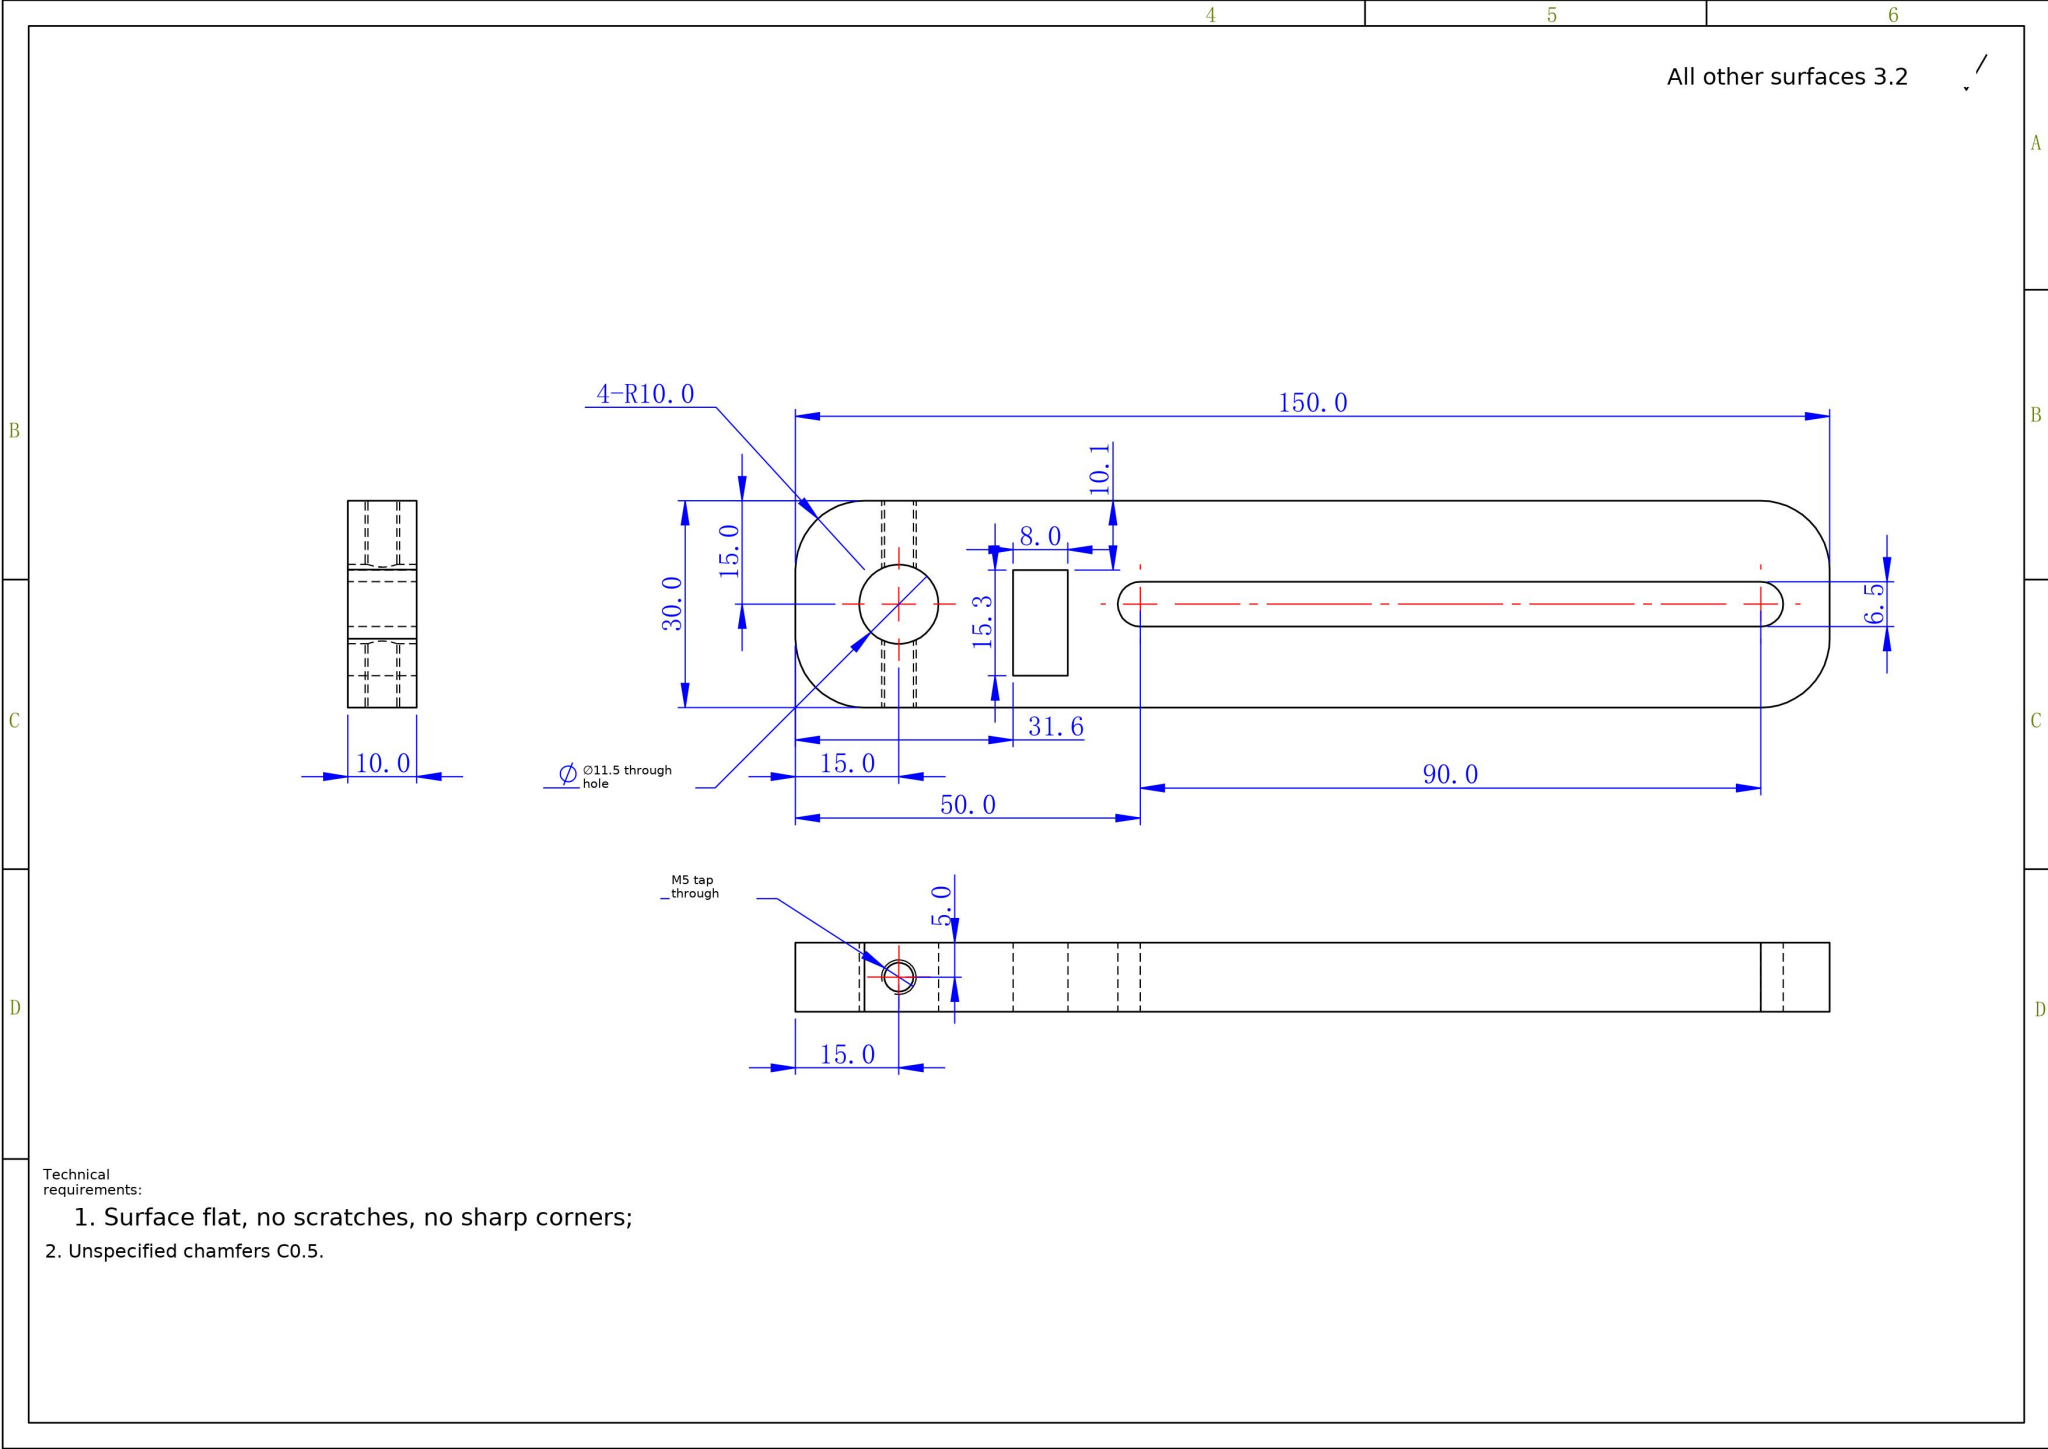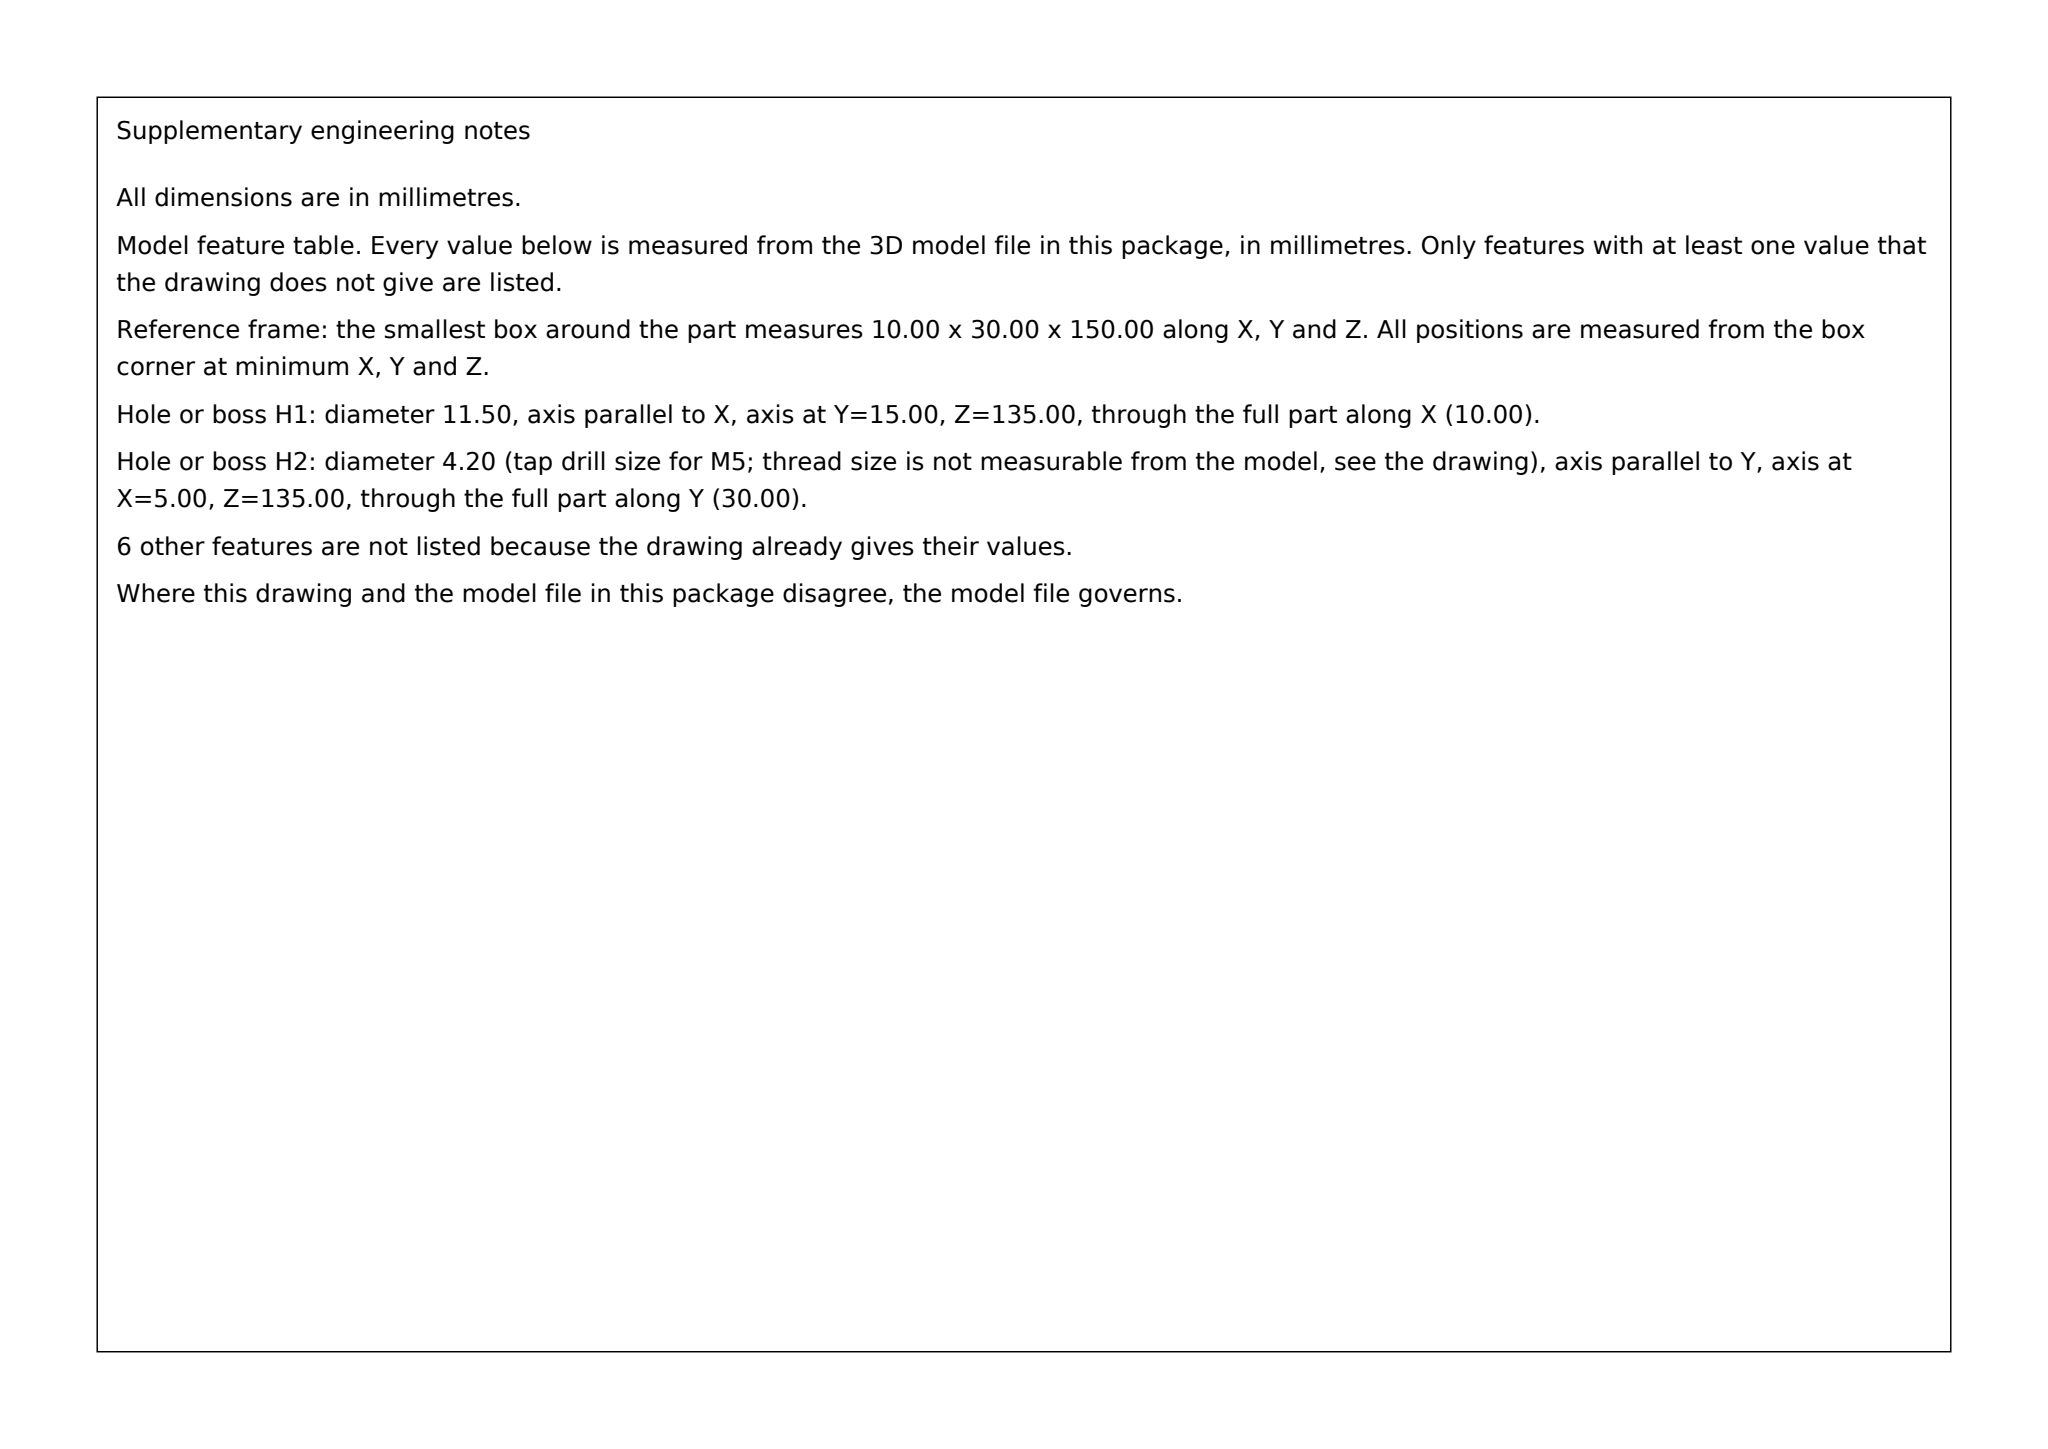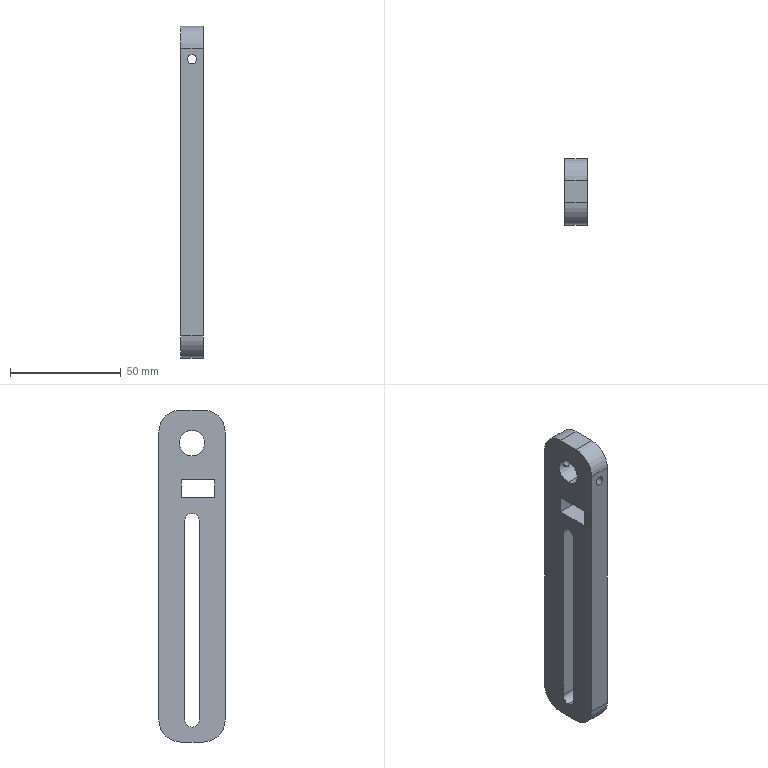Part | SolidWorks | mm | 1 solid | 25 faces | box 10 x 30 x 150 mm | volume 35444 mm3 | cylinder 13 | plane 12 | commonest cylinder face diameters 4.2 x4 20 x4 6.5 x3 11.5 x2